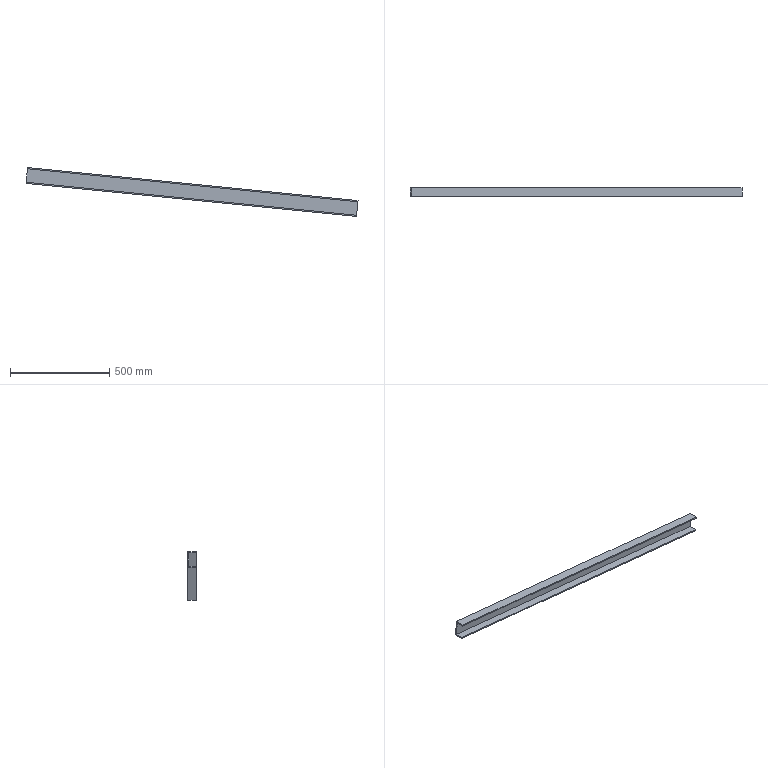Component | NX | UP_FRAME1670_3 | 1 solid | 10 faces | box 1669.69 x 45 x 245.47 mm | volume 1583160 mm3 | plane 10
STEP:
#1=CARTESIAN_POINT('',(0.,0.,0.));
#2=DIRECTION('',(0.,0.,1.));
#3=DIRECTION('',(1.,0.,0.));
#4=AXIS2_PLACEMENT_3D('',#1,#2,#3);
#5=CARTESIAN_POINT('',(-114.972,136.5,534.777));
#6=VERTEX_POINT('',#5);
#7=CARTESIAN_POINT('',(-108.218,136.5,602.441));
#8=VERTEX_POINT('',#7);
#9=CARTESIAN_POINT('',(-114.972,136.5,534.777));
#10=DIRECTION('',(0.09932,0.,0.9951));
#11=VECTOR('',#10,1.);
#12=LINE('',#9,#11);
#13=CARTESIAN_POINT('',(1546.771,136.5,368.913));
#14=DIRECTION('',(0.,-1.,0.));
#15=DIRECTION('',(-0.09932,-0.,-0.9951));
#16=AXIS2_PLACEMENT_3D('',#13,#14,#15);
#17=PLANE('',#16);
#18=CARTESIAN_POINT('',(-0.,-1670.));
#19=DIRECTION('',(-1.,0.));
#20=VECTOR('',#19,1.);
#21=LINE('',#18,#20);
#22=(GEOMETRIC_REPRESENTATION_CONTEXT(2)PARAMETRIC_REPRESENTATION_CONTEXT()REPRESENTATION_CONTEXT('',''));
#23=DEFINITIONAL_REPRESENTATION('',(#21),#22);
#24=PCURVE('',#17,#23);
#25=CARTESIAN_POINT('',(-108.218,136.5,602.441));
#26=DIRECTION('',(0.9951,0.,-0.09932));
#27=DIRECTION('',(0.09932,0.,0.9951));
#28=AXIS2_PLACEMENT_3D('',#25,#26,#27);
#29=PLANE('',#28);
#30=CARTESIAN_POINT('',(-68.,0.));
#31=DIRECTION('',(1.,-0.));
#32=VECTOR('',#31,1.);
#33=LINE('',#30,#32);
#34=(GEOMETRIC_REPRESENTATION_CONTEXT(2)PARAMETRIC_REPRESENTATION_CONTEXT()REPRESENTATION_CONTEXT('',''));
#35=DEFINITIONAL_REPRESENTATION('',(#33),#34);
#36=PCURVE('',#29,#35);
#37=SURFACE_CURVE('',#12,(#24,#36),.PCURVE_S1.);
#38=EDGE_CURVE('',#6,#8,#37,.T.);
#39=ORIENTED_EDGE('',*,*,#38,.F.);
#40=CARTESIAN_POINT('',(1546.771,136.5,368.913));
#41=VERTEX_POINT('',#40);
#42=CARTESIAN_POINT('',(1546.771,136.5,368.913));
#43=DIRECTION('',(-0.9951,0.,0.09932));
#44=VECTOR('',#43,1.);
#45=LINE('',#42,#44);
#46=CARTESIAN_POINT('',(0.,0.));
#47=DIRECTION('',(0.,-1.));
#48=VECTOR('',#47,1.);
#49=LINE('',#46,#48);
#50=(GEOMETRIC_REPRESENTATION_CONTEXT(2)PARAMETRIC_REPRESENTATION_CONTEXT()REPRESENTATION_CONTEXT('',''));
#51=DEFINITIONAL_REPRESENTATION('',(#49),#50);
#52=PCURVE('',#17,#51);
#53=CARTESIAN_POINT('',(1546.771,97.5,368.913));
#54=DIRECTION('',(0.09932,0.,0.9951));
#55=DIRECTION('',(0.,-1.,0.));
#56=AXIS2_PLACEMENT_3D('',#53,#54,#55);
#57=PLANE('',#56);
#58=CARTESIAN_POINT('',(-39.,0.));
#59=DIRECTION('',(0.,-1.));
#60=VECTOR('',#59,1.);
#61=LINE('',#58,#60);
#62=(GEOMETRIC_REPRESENTATION_CONTEXT(2)PARAMETRIC_REPRESENTATION_CONTEXT()REPRESENTATION_CONTEXT('',''));
#63=DEFINITIONAL_REPRESENTATION('',(#61),#62);
#64=PCURVE('',#57,#63);
#65=SURFACE_CURVE('',#45,(#52,#64),.PCURVE_S1.);
#66=EDGE_CURVE('',#41,#6,#65,.T.);
#67=ORIENTED_EDGE('',*,*,#66,.F.);
#68=CARTESIAN_POINT('',(1553.525,136.5,436.577));
#69=VERTEX_POINT('',#68);
#70=CARTESIAN_POINT('',(1546.771,136.5,368.913));
#71=DIRECTION('',(0.09932,0.,0.9951));
#72=VECTOR('',#71,1.);
#73=LINE('',#70,#72);
#74=CARTESIAN_POINT('',(0.,0.));
#75=DIRECTION('',(-1.,0.));
#76=VECTOR('',#75,1.);
#77=LINE('',#74,#76);
#78=(GEOMETRIC_REPRESENTATION_CONTEXT(2)PARAMETRIC_REPRESENTATION_CONTEXT()REPRESENTATION_CONTEXT('',''));
#79=DEFINITIONAL_REPRESENTATION('',(#77),#78);
#80=PCURVE('',#17,#79);
#81=CARTESIAN_POINT('',(1553.525,136.5,436.577));
#82=DIRECTION('',(0.9951,0.,-0.09932));
#83=DIRECTION('',(0.09932,0.,0.9951));
#84=AXIS2_PLACEMENT_3D('',#81,#82,#83);
#85=PLANE('',#84);
#86=CARTESIAN_POINT('',(-68.,0.));
#87=DIRECTION('',(1.,-0.));
#88=VECTOR('',#87,1.);
#89=LINE('',#86,#88);
#90=(GEOMETRIC_REPRESENTATION_CONTEXT(2)PARAMETRIC_REPRESENTATION_CONTEXT()REPRESENTATION_CONTEXT('',''));
#91=DEFINITIONAL_REPRESENTATION('',(#89),#90);
#92=PCURVE('',#85,#91);
#93=SURFACE_CURVE('',#73,(#80,#92),.PCURVE_S1.);
#94=EDGE_CURVE('',#41,#69,#93,.T.);
#95=ORIENTED_EDGE('',*,*,#94,.T.);
#96=CARTESIAN_POINT('',(1553.525,136.5,436.577));
#97=DIRECTION('',(-0.9951,0.,0.09932));
#98=VECTOR('',#97,1.);
#99=LINE('',#96,#98);
#100=CARTESIAN_POINT('',(-68.,0.));
#101=DIRECTION('',(0.,-1.));
#102=VECTOR('',#101,1.);
#103=LINE('',#100,#102);
#104=(GEOMETRIC_REPRESENTATION_CONTEXT(2)PARAMETRIC_REPRESENTATION_CONTEXT()REPRESENTATION_CONTEXT('',''));
#105=DEFINITIONAL_REPRESENTATION('',(#103),#104);
#106=PCURVE('',#17,#105);
#107=CARTESIAN_POINT('',(1553.525,136.5,436.577));
#108=DIRECTION('',(-0.09932,-0.,-0.9951));
#109=DIRECTION('',(-0.,1.,-0.));
#110=AXIS2_PLACEMENT_3D('',#107,#108,#109);
#111=PLANE('',#110);
#112=CARTESIAN_POINT('',(0.,0.));
#113=DIRECTION('',(-0.,-1.));
#114=VECTOR('',#113,1.);
#115=LINE('',#112,#114);
#116=(GEOMETRIC_REPRESENTATION_CONTEXT(2)PARAMETRIC_REPRESENTATION_CONTEXT()REPRESENTATION_CONTEXT('',''));
#117=DEFINITIONAL_REPRESENTATION('',(#115),#116);
#118=PCURVE('',#111,#117);
#119=SURFACE_CURVE('',#99,(#106,#118),.PCURVE_S1.);
#120=EDGE_CURVE('',#69,#8,#119,.T.);
#121=ORIENTED_EDGE('',*,*,#120,.T.);
#122=EDGE_LOOP('',(#39,#67,#95,#121));
#123=FACE_BOUND('',#122,.T.);
#124=ADVANCED_FACE('',(#123),#17,.T.);
#125=CARTESIAN_POINT('',(-108.218,97.5,602.441));
#126=VERTEX_POINT('',#125);
#127=CARTESIAN_POINT('',(-108.218,136.5,602.441));
#128=DIRECTION('',(0.,-1.,0.));
#129=VECTOR('',#128,1.);
#130=LINE('',#127,#129);
#131=CARTESIAN_POINT('',(-0.,-1670.));
#132=DIRECTION('',(-1.,0.));
#133=VECTOR('',#132,1.);
#134=LINE('',#131,#133);
#135=(GEOMETRIC_REPRESENTATION_CONTEXT(2)PARAMETRIC_REPRESENTATION_CONTEXT()REPRESENTATION_CONTEXT('',''));
#136=DEFINITIONAL_REPRESENTATION('',(#134),#135);
#137=PCURVE('',#111,#136);
#138=CARTESIAN_POINT('',(0.,0.));
#139=DIRECTION('',(0.,1.));
#140=VECTOR('',#139,1.);
#141=LINE('',#138,#140);
#142=(GEOMETRIC_REPRESENTATION_CONTEXT(2)PARAMETRIC_REPRESENTATION_CONTEXT()REPRESENTATION_CONTEXT('',''));
#143=DEFINITIONAL_REPRESENTATION('',(#141),#142);
#144=PCURVE('',#29,#143);
#145=SURFACE_CURVE('',#130,(#137,#144),.PCURVE_S1.);
#146=EDGE_CURVE('',#8,#126,#145,.T.);
#147=ORIENTED_EDGE('',*,*,#146,.F.);
#148=ORIENTED_EDGE('',*,*,#120,.F.);
#149=CARTESIAN_POINT('',(1553.525,97.5,436.577));
#150=VERTEX_POINT('',#149);
#151=CARTESIAN_POINT('',(1553.525,136.5,436.577));
#152=DIRECTION('',(0.,-1.,0.));
#153=VECTOR('',#152,1.);
#154=LINE('',#151,#153);
#155=CARTESIAN_POINT('',(0.,0.));
#156=DIRECTION('',(-1.,0.));
#157=VECTOR('',#156,1.);
#158=LINE('',#155,#157);
#159=(GEOMETRIC_REPRESENTATION_CONTEXT(2)PARAMETRIC_REPRESENTATION_CONTEXT()REPRESENTATION_CONTEXT('',''));
#160=DEFINITIONAL_REPRESENTATION('',(#158),#159);
#161=PCURVE('',#111,#160);
#162=CARTESIAN_POINT('',(0.,0.));
#163=DIRECTION('',(0.,1.));
#164=VECTOR('',#163,1.);
#165=LINE('',#162,#164);
#166=(GEOMETRIC_REPRESENTATION_CONTEXT(2)PARAMETRIC_REPRESENTATION_CONTEXT()REPRESENTATION_CONTEXT('',''));
#167=DEFINITIONAL_REPRESENTATION('',(#165),#166);
#168=PCURVE('',#85,#167);
#169=SURFACE_CURVE('',#154,(#161,#168),.PCURVE_S1.);
#170=EDGE_CURVE('',#69,#150,#169,.T.);
#171=ORIENTED_EDGE('',*,*,#170,.T.);
#172=CARTESIAN_POINT('',(1553.525,97.5,436.577));
#173=DIRECTION('',(-0.9951,0.,0.09932));
#174=VECTOR('',#173,1.);
#175=LINE('',#172,#174);
#176=CARTESIAN_POINT('',(-39.,-0.));
#177=DIRECTION('',(-0.,-1.));
#178=VECTOR('',#177,1.);
#179=LINE('',#176,#178);
#180=(GEOMETRIC_REPRESENTATION_CONTEXT(2)PARAMETRIC_REPRESENTATION_CONTEXT()REPRESENTATION_CONTEXT('',''));
#181=DEFINITIONAL_REPRESENTATION('',(#179),#180);
#182=PCURVE('',#111,#181);
#183=CARTESIAN_POINT('',(1553.525,97.5,436.577));
#184=DIRECTION('',(0.,-1.,0.));
#185=DIRECTION('',(-0.09932,0.,-0.9951));
#186=AXIS2_PLACEMENT_3D('',#183,#184,#185);
#187=PLANE('',#186);
#188=CARTESIAN_POINT('',(0.,0.));
#189=DIRECTION('',(0.,-1.));
#190=VECTOR('',#189,1.);
#191=LINE('',#188,#190);
#192=(GEOMETRIC_REPRESENTATION_CONTEXT(2)PARAMETRIC_REPRESENTATION_CONTEXT()REPRESENTATION_CONTEXT('',''));
#193=DEFINITIONAL_REPRESENTATION('',(#191),#192);
#194=PCURVE('',#187,#193);
#195=SURFACE_CURVE('',#175,(#182,#194),.PCURVE_S1.);
#196=EDGE_CURVE('',#150,#126,#195,.T.);
#197=ORIENTED_EDGE('',*,*,#196,.T.);
#198=EDGE_LOOP('',(#147,#148,#171,#197));
#199=FACE_BOUND('',#198,.T.);
#200=ADVANCED_FACE('',(#199),#111,.T.);
#201=CARTESIAN_POINT('',(-107.622,97.5,608.412));
#202=VERTEX_POINT('',#201);
#203=CARTESIAN_POINT('',(-108.218,97.5,602.441));
#204=DIRECTION('',(0.09932,0.,0.9951));
#205=VECTOR('',#204,1.);
#206=LINE('',#203,#205);
#207=CARTESIAN_POINT('',(0.,-1670.));
#208=DIRECTION('',(-1.,0.));
#209=VECTOR('',#208,1.);
#210=LINE('',#207,#209);
#211=(GEOMETRIC_REPRESENTATION_CONTEXT(2)PARAMETRIC_REPRESENTATION_CONTEXT()REPRESENTATION_CONTEXT('',''));
#212=DEFINITIONAL_REPRESENTATION('',(#210),#211);
#213=PCURVE('',#187,#212);
#214=CARTESIAN_POINT('',(0.,39.));
#215=DIRECTION('',(1.,0.));
#216=VECTOR('',#215,1.);
#217=LINE('',#214,#216);
#218=(GEOMETRIC_REPRESENTATION_CONTEXT(2)PARAMETRIC_REPRESENTATION_CONTEXT()REPRESENTATION_CONTEXT('',''));
#219=DEFINITIONAL_REPRESENTATION('',(#217),#218);
#220=PCURVE('',#29,#219);
#221=SURFACE_CURVE('',#206,(#213,#220),.PCURVE_S1.);
#222=EDGE_CURVE('',#126,#202,#221,.T.);
#223=ORIENTED_EDGE('',*,*,#222,.F.);
#224=ORIENTED_EDGE('',*,*,#196,.F.);
#225=CARTESIAN_POINT('',(1554.12,97.5,442.548));
#226=VERTEX_POINT('',#225);
#227=CARTESIAN_POINT('',(1553.525,97.5,436.577));
#228=DIRECTION('',(0.09932,0.,0.9951));
#229=VECTOR('',#228,1.);
#230=LINE('',#227,#229);
#231=CARTESIAN_POINT('',(0.,0.));
#232=DIRECTION('',(-1.,0.));
#233=VECTOR('',#232,1.);
#234=LINE('',#231,#233);
#235=(GEOMETRIC_REPRESENTATION_CONTEXT(2)PARAMETRIC_REPRESENTATION_CONTEXT()REPRESENTATION_CONTEXT('',''));
#236=DEFINITIONAL_REPRESENTATION('',(#234),#235);
#237=PCURVE('',#187,#236);
#238=CARTESIAN_POINT('',(0.,39.));
#239=DIRECTION('',(1.,0.));
#240=VECTOR('',#239,1.);
#241=LINE('',#238,#240);
#242=(GEOMETRIC_REPRESENTATION_CONTEXT(2)PARAMETRIC_REPRESENTATION_CONTEXT()REPRESENTATION_CONTEXT('',''));
#243=DEFINITIONAL_REPRESENTATION('',(#241),#242);
#244=PCURVE('',#85,#243);
#245=SURFACE_CURVE('',#230,(#237,#244),.PCURVE_S1.);
#246=EDGE_CURVE('',#150,#226,#245,.T.);
#247=ORIENTED_EDGE('',*,*,#246,.T.);
#248=CARTESIAN_POINT('',(1554.12,97.5,442.548));
#249=DIRECTION('',(-0.9951,0.,0.09932));
#250=VECTOR('',#249,1.);
#251=LINE('',#248,#250);
#252=CARTESIAN_POINT('',(-6.,-0.));
#253=DIRECTION('',(0.,-1.));
#254=VECTOR('',#253,1.);
#255=LINE('',#252,#254);
#256=(GEOMETRIC_REPRESENTATION_CONTEXT(2)PARAMETRIC_REPRESENTATION_CONTEXT()REPRESENTATION_CONTEXT('',''));
#257=DEFINITIONAL_REPRESENTATION('',(#255),#256);
#258=PCURVE('',#187,#257);
#259=CARTESIAN_POINT('',(1554.12,97.5,442.548));
#260=DIRECTION('',(0.09932,0.,0.9951));
#261=DIRECTION('',(-0.9951,0.,0.09932));
#262=AXIS2_PLACEMENT_3D('',#259,#260,#261);
#263=PLANE('',#262);
#264=CARTESIAN_POINT('',(0.,0.));
#265=DIRECTION('',(1.,0.));
#266=VECTOR('',#265,1.);
#267=LINE('',#264,#266);
#268=(GEOMETRIC_REPRESENTATION_CONTEXT(2)PARAMETRIC_REPRESENTATION_CONTEXT()REPRESENTATION_CONTEXT('',''));
#269=DEFINITIONAL_REPRESENTATION('',(#267),#268);
#270=PCURVE('',#263,#269);
#271=SURFACE_CURVE('',#251,(#258,#270),.PCURVE_S1.);
#272=EDGE_CURVE('',#226,#202,#271,.T.);
#273=ORIENTED_EDGE('',*,*,#272,.T.);
#274=EDGE_LOOP('',(#223,#224,#247,#273));
#275=FACE_BOUND('',#274,.T.);
#276=ADVANCED_FACE('',(#275),#187,.T.);
#277=CARTESIAN_POINT('',(-107.622,142.5,608.412));
#278=VERTEX_POINT('',#277);
#279=CARTESIAN_POINT('',(-107.622,97.5,608.412));
#280=DIRECTION('',(0.,1.,0.));
#281=VECTOR('',#280,1.);
#282=LINE('',#279,#281);
#283=CARTESIAN_POINT('',(1670.,0.));
#284=DIRECTION('',(0.,-1.));
#285=VECTOR('',#284,1.);
#286=LINE('',#283,#285);
#287=(GEOMETRIC_REPRESENTATION_CONTEXT(2)PARAMETRIC_REPRESENTATION_CONTEXT()REPRESENTATION_CONTEXT('',''));
#288=DEFINITIONAL_REPRESENTATION('',(#286),#287);
#289=PCURVE('',#263,#288);
#290=CARTESIAN_POINT('',(6.,39.));
#291=DIRECTION('',(0.,-1.));
#292=VECTOR('',#291,1.);
#293=LINE('',#290,#292);
#294=(GEOMETRIC_REPRESENTATION_CONTEXT(2)PARAMETRIC_REPRESENTATION_CONTEXT()REPRESENTATION_CONTEXT('',''));
#295=DEFINITIONAL_REPRESENTATION('',(#293),#294);
#296=PCURVE('',#29,#295);
#297=SURFACE_CURVE('',#282,(#289,#296),.PCURVE_S1.);
#298=EDGE_CURVE('',#202,#278,#297,.T.);
#299=ORIENTED_EDGE('',*,*,#298,.F.);
#300=ORIENTED_EDGE('',*,*,#272,.F.);
#301=CARTESIAN_POINT('',(1554.12,142.5,442.548));
#302=VERTEX_POINT('',#301);
#303=CARTESIAN_POINT('',(1554.12,97.5,442.548));
#304=DIRECTION('',(0.,1.,0.));
#305=VECTOR('',#304,1.);
#306=LINE('',#303,#305);
#307=CARTESIAN_POINT('',(0.,0.));
#308=DIRECTION('',(0.,-1.));
#309=VECTOR('',#308,1.);
#310=LINE('',#307,#309);
#311=(GEOMETRIC_REPRESENTATION_CONTEXT(2)PARAMETRIC_REPRESENTATION_CONTEXT()REPRESENTATION_CONTEXT('',''));
#312=DEFINITIONAL_REPRESENTATION('',(#310),#311);
#313=PCURVE('',#263,#312);
#314=CARTESIAN_POINT('',(6.,39.));
#315=DIRECTION('',(0.,-1.));
#316=VECTOR('',#315,1.);
#317=LINE('',#314,#316);
#318=(GEOMETRIC_REPRESENTATION_CONTEXT(2)PARAMETRIC_REPRESENTATION_CONTEXT()REPRESENTATION_CONTEXT('',''));
#319=DEFINITIONAL_REPRESENTATION('',(#317),#318);
#320=PCURVE('',#85,#319);
#321=SURFACE_CURVE('',#306,(#313,#320),.PCURVE_S1.);
#322=EDGE_CURVE('',#226,#302,#321,.T.);
#323=ORIENTED_EDGE('',*,*,#322,.T.);
#324=CARTESIAN_POINT('',(1554.12,142.5,442.548));
#325=DIRECTION('',(-0.9951,0.,0.09932));
#326=VECTOR('',#325,1.);
#327=LINE('',#324,#326);
#328=CARTESIAN_POINT('',(0.,-45.));
#329=DIRECTION('',(1.,0.));
#330=VECTOR('',#329,1.);
#331=LINE('',#328,#330);
#332=(GEOMETRIC_REPRESENTATION_CONTEXT(2)PARAMETRIC_REPRESENTATION_CONTEXT()REPRESENTATION_CONTEXT('',''));
#333=DEFINITIONAL_REPRESENTATION('',(#331),#332);
#334=PCURVE('',#263,#333);
#335=CARTESIAN_POINT('',(1554.12,142.5,442.548));
#336=DIRECTION('',(-0.,1.,-0.));
#337=DIRECTION('',(0.09932,0.,0.9951));
#338=AXIS2_PLACEMENT_3D('',#335,#336,#337);
#339=PLANE('',#338);
#340=CARTESIAN_POINT('',(0.,0.));
#341=DIRECTION('',(0.,-1.));
#342=VECTOR('',#341,1.);
#343=LINE('',#340,#342);
#344=(GEOMETRIC_REPRESENTATION_CONTEXT(2)PARAMETRIC_REPRESENTATION_CONTEXT()REPRESENTATION_CONTEXT('',''));
#345=DEFINITIONAL_REPRESENTATION('',(#343),#344);
#346=PCURVE('',#339,#345);
#347=SURFACE_CURVE('',#327,(#334,#346),.PCURVE_S1.);
#348=EDGE_CURVE('',#302,#278,#347,.T.);
#349=ORIENTED_EDGE('',*,*,#348,.T.);
#350=EDGE_LOOP('',(#299,#300,#323,#349));
#351=FACE_BOUND('',#350,.T.);
#352=ADVANCED_FACE('',(#351),#263,.T.);
#353=CARTESIAN_POINT('',(-115.568,142.5,528.807));
#354=VERTEX_POINT('',#353);
#355=CARTESIAN_POINT('',(-107.622,142.5,608.412));
#356=DIRECTION('',(-0.09932,-0.,-0.9951));
#357=VECTOR('',#356,1.);
#358=LINE('',#355,#357);
#359=CARTESIAN_POINT('',(0.,-1670.));
#360=DIRECTION('',(-1.,0.));
#361=VECTOR('',#360,1.);
#362=LINE('',#359,#361);
#363=(GEOMETRIC_REPRESENTATION_CONTEXT(2)PARAMETRIC_REPRESENTATION_CONTEXT()REPRESENTATION_CONTEXT('',''));
#364=DEFINITIONAL_REPRESENTATION('',(#362),#363);
#365=PCURVE('',#339,#364);
#366=CARTESIAN_POINT('',(6.,-6.));
#367=DIRECTION('',(-1.,0.));
#368=VECTOR('',#367,1.);
#369=LINE('',#366,#368);
#370=(GEOMETRIC_REPRESENTATION_CONTEXT(2)PARAMETRIC_REPRESENTATION_CONTEXT()REPRESENTATION_CONTEXT('',''));
#371=DEFINITIONAL_REPRESENTATION('',(#369),#370);
#372=PCURVE('',#29,#371);
#373=SURFACE_CURVE('',#358,(#365,#372),.PCURVE_S1.);
#374=EDGE_CURVE('',#278,#354,#373,.T.);
#375=ORIENTED_EDGE('',*,*,#374,.F.);
#376=ORIENTED_EDGE('',*,*,#348,.F.);
#377=CARTESIAN_POINT('',(1546.175,142.5,362.943));
#378=VERTEX_POINT('',#377);
#379=CARTESIAN_POINT('',(1554.12,142.5,442.548));
#380=DIRECTION('',(-0.09932,-0.,-0.9951));
#381=VECTOR('',#380,1.);
#382=LINE('',#379,#381);
#383=CARTESIAN_POINT('',(0.,0.));
#384=DIRECTION('',(-1.,0.));
#385=VECTOR('',#384,1.);
#386=LINE('',#383,#385);
#387=(GEOMETRIC_REPRESENTATION_CONTEXT(2)PARAMETRIC_REPRESENTATION_CONTEXT()REPRESENTATION_CONTEXT('',''));
#388=DEFINITIONAL_REPRESENTATION('',(#386),#387);
#389=PCURVE('',#339,#388);
#390=CARTESIAN_POINT('',(6.,-6.));
#391=DIRECTION('',(-1.,0.));
#392=VECTOR('',#391,1.);
#393=LINE('',#390,#392);
#394=(GEOMETRIC_REPRESENTATION_CONTEXT(2)PARAMETRIC_REPRESENTATION_CONTEXT()REPRESENTATION_CONTEXT('',''));
#395=DEFINITIONAL_REPRESENTATION('',(#393),#394);
#396=PCURVE('',#85,#395);
#397=SURFACE_CURVE('',#382,(#389,#396),.PCURVE_S1.);
#398=EDGE_CURVE('',#302,#378,#397,.T.);
#399=ORIENTED_EDGE('',*,*,#398,.T.);
#400=CARTESIAN_POINT('',(1546.175,142.5,362.943));
#401=DIRECTION('',(-0.9951,0.,0.09932));
#402=VECTOR('',#401,1.);
#403=LINE('',#400,#402);
#404=CARTESIAN_POINT('',(-80.,0.));
#405=DIRECTION('',(0.,-1.));
#406=VECTOR('',#405,1.);
#407=LINE('',#404,#406);
#408=(GEOMETRIC_REPRESENTATION_CONTEXT(2)PARAMETRIC_REPRESENTATION_CONTEXT()REPRESENTATION_CONTEXT('',''));
#409=DEFINITIONAL_REPRESENTATION('',(#407),#408);
#410=PCURVE('',#339,#409);
#411=CARTESIAN_POINT('',(1546.175,142.5,362.943));
#412=DIRECTION('',(-0.09932,0.,-0.9951));
#413=DIRECTION('',(0.9951,0.,-0.09932));
#414=AXIS2_PLACEMENT_3D('',#411,#412,#413);
#415=PLANE('',#414);
#416=CARTESIAN_POINT('',(0.,0.));
#417=DIRECTION('',(-1.,0.));
#418=VECTOR('',#417,1.);
#419=LINE('',#416,#418);
#420=(GEOMETRIC_REPRESENTATION_CONTEXT(2)PARAMETRIC_REPRESENTATION_CONTEXT()REPRESENTATION_CONTEXT('',''));
#421=DEFINITIONAL_REPRESENTATION('',(#419),#420);
#422=PCURVE('',#415,#421);
#423=SURFACE_CURVE('',#403,(#410,#422),.PCURVE_S1.);
#424=EDGE_CURVE('',#378,#354,#423,.T.);
#425=ORIENTED_EDGE('',*,*,#424,.T.);
#426=EDGE_LOOP('',(#375,#376,#399,#425));
#427=FACE_BOUND('',#426,.T.);
#428=ADVANCED_FACE('',(#427),#339,.T.);
#429=CARTESIAN_POINT('',(-115.568,97.5,528.807));
#430=VERTEX_POINT('',#429);
#431=CARTESIAN_POINT('',(-115.568,142.5,528.807));
#432=DIRECTION('',(0.,-1.,0.));
#433=VECTOR('',#432,1.);
#434=LINE('',#431,#433);
#435=CARTESIAN_POINT('',(-1670.,0.));
#436=DIRECTION('',(0.,1.));
#437=VECTOR('',#436,1.);
#438=LINE('',#435,#437);
#439=(GEOMETRIC_REPRESENTATION_CONTEXT(2)PARAMETRIC_REPRESENTATION_CONTEXT()REPRESENTATION_CONTEXT('',''));
#440=DEFINITIONAL_REPRESENTATION('',(#438),#439);
#441=PCURVE('',#415,#440);
#442=CARTESIAN_POINT('',(-74.,-6.));
#443=DIRECTION('',(0.,1.));
#444=VECTOR('',#443,1.);
#445=LINE('',#442,#444);
#446=(GEOMETRIC_REPRESENTATION_CONTEXT(2)PARAMETRIC_REPRESENTATION_CONTEXT()REPRESENTATION_CONTEXT('',''));
#447=DEFINITIONAL_REPRESENTATION('',(#445),#446);
#448=PCURVE('',#29,#447);
#449=SURFACE_CURVE('',#434,(#441,#448),.PCURVE_S1.);
#450=EDGE_CURVE('',#354,#430,#449,.T.);
#451=ORIENTED_EDGE('',*,*,#450,.F.);
#452=ORIENTED_EDGE('',*,*,#424,.F.);
#453=CARTESIAN_POINT('',(1546.175,97.5,362.943));
#454=VERTEX_POINT('',#453);
#455=CARTESIAN_POINT('',(1546.175,142.5,362.943));
#456=DIRECTION('',(0.,-1.,0.));
#457=VECTOR('',#456,1.);
#458=LINE('',#455,#457);
#459=CARTESIAN_POINT('',(0.,0.));
#460=DIRECTION('',(0.,1.));
#461=VECTOR('',#460,1.);
#462=LINE('',#459,#461);
#463=(GEOMETRIC_REPRESENTATION_CONTEXT(2)PARAMETRIC_REPRESENTATION_CONTEXT()REPRESENTATION_CONTEXT('',''));
#464=DEFINITIONAL_REPRESENTATION('',(#462),#463);
#465=PCURVE('',#415,#464);
#466=CARTESIAN_POINT('',(-74.,-6.));
#467=DIRECTION('',(0.,1.));
#468=VECTOR('',#467,1.);
#469=LINE('',#466,#468);
#470=(GEOMETRIC_REPRESENTATION_CONTEXT(2)PARAMETRIC_REPRESENTATION_CONTEXT()REPRESENTATION_CONTEXT('',''));
#471=DEFINITIONAL_REPRESENTATION('',(#469),#470);
#472=PCURVE('',#85,#471);
#473=SURFACE_CURVE('',#458,(#465,#472),.PCURVE_S1.);
#474=EDGE_CURVE('',#378,#454,#473,.T.);
#475=ORIENTED_EDGE('',*,*,#474,.T.);
#476=CARTESIAN_POINT('',(1546.175,97.5,362.943));
#477=DIRECTION('',(-0.9951,0.,0.09932));
#478=VECTOR('',#477,1.);
#479=LINE('',#476,#478);
#480=CARTESIAN_POINT('',(0.,45.));
#481=DIRECTION('',(-1.,0.));
#482=VECTOR('',#481,1.);
#483=LINE('',#480,#482);
#484=(GEOMETRIC_REPRESENTATION_CONTEXT(2)PARAMETRIC_REPRESENTATION_CONTEXT()REPRESENTATION_CONTEXT('',''));
#485=DEFINITIONAL_REPRESENTATION('',(#483),#484);
#486=PCURVE('',#415,#485);
#487=CARTESIAN_POINT('',(1546.175,97.5,362.943));
#488=DIRECTION('',(0.,-1.,0.));
#489=DIRECTION('',(-0.09932,-0.,-0.9951));
#490=AXIS2_PLACEMENT_3D('',#487,#488,#489);
#491=PLANE('',#490);
#492=CARTESIAN_POINT('',(0.,0.));
#493=DIRECTION('',(0.,-1.));
#494=VECTOR('',#493,1.);
#495=LINE('',#492,#494);
#496=(GEOMETRIC_REPRESENTATION_CONTEXT(2)PARAMETRIC_REPRESENTATION_CONTEXT()REPRESENTATION_CONTEXT('',''));
#497=DEFINITIONAL_REPRESENTATION('',(#495),#496);
#498=PCURVE('',#491,#497);
#499=SURFACE_CURVE('',#479,(#486,#498),.PCURVE_S1.);
#500=EDGE_CURVE('',#454,#430,#499,.T.);
#501=ORIENTED_EDGE('',*,*,#500,.T.);
#502=EDGE_LOOP('',(#451,#452,#475,#501));
#503=FACE_BOUND('',#502,.T.);
#504=ADVANCED_FACE('',(#503),#415,.T.);
#505=CARTESIAN_POINT('',(-114.972,97.5,534.777));
#506=VERTEX_POINT('',#505);
#507=CARTESIAN_POINT('',(-115.568,97.5,528.807));
#508=DIRECTION('',(0.09932,0.,0.9951));
#509=VECTOR('',#508,1.);
#510=LINE('',#507,#509);
#511=CARTESIAN_POINT('',(-0.,-1670.));
#512=DIRECTION('',(-1.,0.));
#513=VECTOR('',#512,1.);
#514=LINE('',#511,#513);
#515=(GEOMETRIC_REPRESENTATION_CONTEXT(2)PARAMETRIC_REPRESENTATION_CONTEXT()REPRESENTATION_CONTEXT('',''));
#516=DEFINITIONAL_REPRESENTATION('',(#514),#515);
#517=PCURVE('',#491,#516);
#518=CARTESIAN_POINT('',(-74.,39.));
#519=DIRECTION('',(1.,-0.));
#520=VECTOR('',#519,1.);
#521=LINE('',#518,#520);
#522=(GEOMETRIC_REPRESENTATION_CONTEXT(2)PARAMETRIC_REPRESENTATION_CONTEXT()REPRESENTATION_CONTEXT('',''));
#523=DEFINITIONAL_REPRESENTATION('',(#521),#522);
#524=PCURVE('',#29,#523);
#525=SURFACE_CURVE('',#510,(#517,#524),.PCURVE_S1.);
#526=EDGE_CURVE('',#430,#506,#525,.T.);
#527=ORIENTED_EDGE('',*,*,#526,.F.);
#528=ORIENTED_EDGE('',*,*,#500,.F.);
#529=CARTESIAN_POINT('',(1546.771,97.5,368.913));
#530=VERTEX_POINT('',#529);
#531=CARTESIAN_POINT('',(1546.175,97.5,362.943));
#532=DIRECTION('',(0.09932,0.,0.9951));
#533=VECTOR('',#532,1.);
#534=LINE('',#531,#533);
#535=CARTESIAN_POINT('',(0.,0.));
#536=DIRECTION('',(-1.,0.));
#537=VECTOR('',#536,1.);
#538=LINE('',#535,#537);
#539=(GEOMETRIC_REPRESENTATION_CONTEXT(2)PARAMETRIC_REPRESENTATION_CONTEXT()REPRESENTATION_CONTEXT('',''));
#540=DEFINITIONAL_REPRESENTATION('',(#538),#539);
#541=PCURVE('',#491,#540);
#542=CARTESIAN_POINT('',(-74.,39.));
#543=DIRECTION('',(1.,-0.));
#544=VECTOR('',#543,1.);
#545=LINE('',#542,#544);
#546=(GEOMETRIC_REPRESENTATION_CONTEXT(2)PARAMETRIC_REPRESENTATION_CONTEXT()REPRESENTATION_CONTEXT('',''));
#547=DEFINITIONAL_REPRESENTATION('',(#545),#546);
#548=PCURVE('',#85,#547);
#549=SURFACE_CURVE('',#534,(#541,#548),.PCURVE_S1.);
#550=EDGE_CURVE('',#454,#530,#549,.T.);
#551=ORIENTED_EDGE('',*,*,#550,.T.);
#552=CARTESIAN_POINT('',(1546.771,97.5,368.913));
#553=DIRECTION('',(-0.9951,0.,0.09932));
#554=VECTOR('',#553,1.);
#555=LINE('',#552,#554);
#556=CARTESIAN_POINT('',(-6.,-0.));
#557=DIRECTION('',(0.,-1.));
#558=VECTOR('',#557,1.);
#559=LINE('',#556,#558);
#560=(GEOMETRIC_REPRESENTATION_CONTEXT(2)PARAMETRIC_REPRESENTATION_CONTEXT()REPRESENTATION_CONTEXT('',''));
#561=DEFINITIONAL_REPRESENTATION('',(#559),#560);
#562=PCURVE('',#491,#561);
#563=CARTESIAN_POINT('',(0.,0.));
#564=DIRECTION('',(0.,-1.));
#565=VECTOR('',#564,1.);
#566=LINE('',#563,#565);
#567=(GEOMETRIC_REPRESENTATION_CONTEXT(2)PARAMETRIC_REPRESENTATION_CONTEXT()REPRESENTATION_CONTEXT('',''));
#568=DEFINITIONAL_REPRESENTATION('',(#566),#567);
#569=PCURVE('',#57,#568);
#570=SURFACE_CURVE('',#555,(#562,#569),.PCURVE_S1.);
#571=EDGE_CURVE('',#530,#506,#570,.T.);
#572=ORIENTED_EDGE('',*,*,#571,.T.);
#573=EDGE_LOOP('',(#527,#528,#551,#572));
#574=FACE_BOUND('',#573,.T.);
#575=ADVANCED_FACE('',(#574),#491,.T.);
#576=CARTESIAN_POINT('',(-114.972,97.5,534.777));
#577=DIRECTION('',(-0.,1.,-0.));
#578=VECTOR('',#577,1.);
#579=LINE('',#576,#578);
#580=CARTESIAN_POINT('',(0.,-1670.));
#581=DIRECTION('',(-1.,-0.));
#582=VECTOR('',#581,1.);
#583=LINE('',#580,#582);
#584=(GEOMETRIC_REPRESENTATION_CONTEXT(2)PARAMETRIC_REPRESENTATION_CONTEXT()REPRESENTATION_CONTEXT('',''));
#585=DEFINITIONAL_REPRESENTATION('',(#583),#584);
#586=PCURVE('',#57,#585);
#587=CARTESIAN_POINT('',(-68.,39.));
#588=DIRECTION('',(-0.,-1.));
#589=VECTOR('',#588,1.);
#590=LINE('',#587,#589);
#591=(GEOMETRIC_REPRESENTATION_CONTEXT(2)PARAMETRIC_REPRESENTATION_CONTEXT()REPRESENTATION_CONTEXT('',''));
#592=DEFINITIONAL_REPRESENTATION('',(#590),#591);
#593=PCURVE('',#29,#592);
#594=SURFACE_CURVE('',#579,(#586,#593),.PCURVE_S1.);
#595=EDGE_CURVE('',#506,#6,#594,.T.);
#596=ORIENTED_EDGE('',*,*,#595,.F.);
#597=ORIENTED_EDGE('',*,*,#571,.F.);
#598=CARTESIAN_POINT('',(1546.771,97.5,368.913));
#599=DIRECTION('',(-0.,1.,-0.));
#600=VECTOR('',#599,1.);
#601=LINE('',#598,#600);
#602=CARTESIAN_POINT('',(0.,0.));
#603=DIRECTION('',(-1.,-0.));
#604=VECTOR('',#603,1.);
#605=LINE('',#602,#604);
#606=(GEOMETRIC_REPRESENTATION_CONTEXT(2)PARAMETRIC_REPRESENTATION_CONTEXT()REPRESENTATION_CONTEXT('',''));
#607=DEFINITIONAL_REPRESENTATION('',(#605),#606);
#608=PCURVE('',#57,#607);
#609=CARTESIAN_POINT('',(-68.,39.));
#610=DIRECTION('',(-0.,-1.));
#611=VECTOR('',#610,1.);
#612=LINE('',#609,#611);
#613=(GEOMETRIC_REPRESENTATION_CONTEXT(2)PARAMETRIC_REPRESENTATION_CONTEXT()REPRESENTATION_CONTEXT('',''));
#614=DEFINITIONAL_REPRESENTATION('',(#612),#613);
#615=PCURVE('',#85,#614);
#616=SURFACE_CURVE('',#601,(#608,#615),.PCURVE_S1.);
#617=EDGE_CURVE('',#530,#41,#616,.T.);
#618=ORIENTED_EDGE('',*,*,#617,.T.);
#619=ORIENTED_EDGE('',*,*,#66,.T.);
#620=EDGE_LOOP('',(#596,#597,#618,#619));
#621=FACE_BOUND('',#620,.T.);
#622=ADVANCED_FACE('',(#621),#57,.T.);
#623=ORIENTED_EDGE('',*,*,#94,.F.);
#624=ORIENTED_EDGE('',*,*,#617,.F.);
#625=ORIENTED_EDGE('',*,*,#550,.F.);
#626=ORIENTED_EDGE('',*,*,#474,.F.);
#627=ORIENTED_EDGE('',*,*,#398,.F.);
#628=ORIENTED_EDGE('',*,*,#322,.F.);
#629=ORIENTED_EDGE('',*,*,#246,.F.);
#630=ORIENTED_EDGE('',*,*,#170,.F.);
#631=EDGE_LOOP('',(#623,#624,#625,#626,#627,#628,#629,#630));
#632=FACE_BOUND('',#631,.T.);
#633=ADVANCED_FACE('',(#632),#85,.T.);
#634=ORIENTED_EDGE('',*,*,#38,.T.);
#635=ORIENTED_EDGE('',*,*,#146,.T.);
#636=ORIENTED_EDGE('',*,*,#222,.T.);
#637=ORIENTED_EDGE('',*,*,#298,.T.);
#638=ORIENTED_EDGE('',*,*,#374,.T.);
#639=ORIENTED_EDGE('',*,*,#450,.T.);
#640=ORIENTED_EDGE('',*,*,#526,.T.);
#641=ORIENTED_EDGE('',*,*,#595,.T.);
#642=EDGE_LOOP('',(#634,#635,#636,#637,#638,#639,#640,#641));
#643=FACE_BOUND('',#642,.T.);
#644=ADVANCED_FACE('',(#643),#29,.F.);
#645=CLOSED_SHELL('',(#124,#200,#276,#352,#428,#504,#575,#622,#633,#644));
#646=MANIFOLD_SOLID_BREP('',#645);
#647=(LENGTH_UNIT()NAMED_UNIT(*)SI_UNIT(.MILLI.,.METRE.));
#648=UNCERTAINTY_MEASURE_WITH_UNIT(LENGTH_MEASURE(0.0000001),#647,'','');
#649=(NAMED_UNIT(*)PLANE_ANGLE_UNIT()SI_UNIT($,.RADIAN.));
#650=(NAMED_UNIT(*)SI_UNIT($,.STERADIAN.)SOLID_ANGLE_UNIT());
#651=(GEOMETRIC_REPRESENTATION_CONTEXT(3)GLOBAL_UNCERTAINTY_ASSIGNED_CONTEXT((#648))GLOBAL_UNIT_ASSIGNED_CONTEXT((#647,#649,#650))REPRESENTATION_CONTEXT('',''));
#652=ADVANCED_BREP_SHAPE_REPRESENTATION('',(#4,#646),#651);